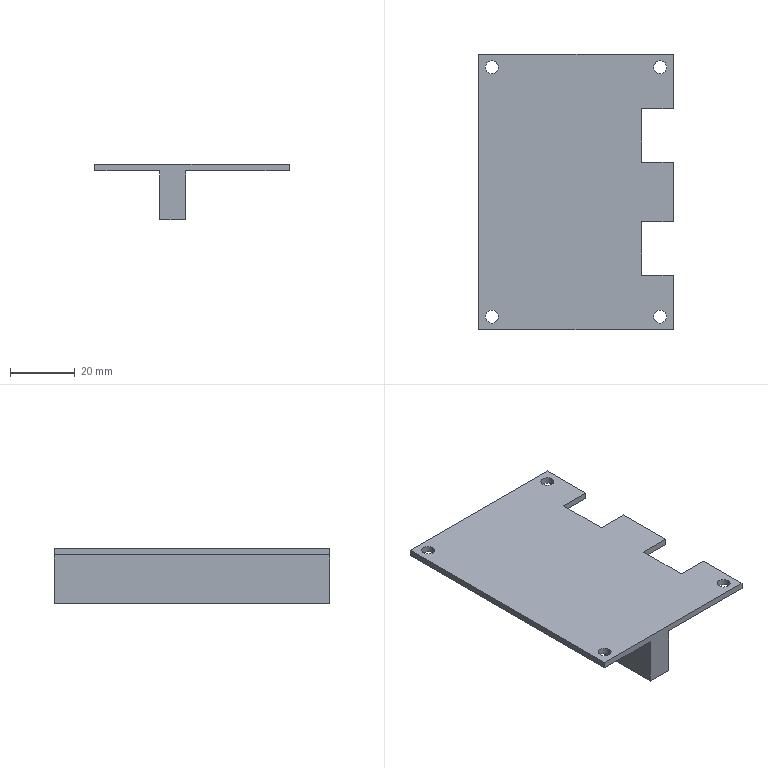Component | SolidWorks | WheelAssembly2-1_CoverPlate-1 | 1 solid | 26 faces | box 60 x 85 x 17 mm | volume 19659 mm3 | plane 18 | cylinder 8 | commonest cylinder face diameters 4 x8
STEP:
#1=CARTESIAN_POINT('',(-12.835,-1.516,-13.581));
#2=VERTEX_POINT('',#1);
#3=CARTESIAN_POINT('',(-12.677,-1.516,-13.581));
#4=VERTEX_POINT('',#3);
#5=CARTESIAN_POINT('',(-12.756,-1.516,-13.581));
#6=DIRECTION('',(0.,-0.,1.));
#7=DIRECTION('',(-1.,0.,0.));
#8=AXIS2_PLACEMENT_3D('',#5,#6,#7);
#9=CIRCLE('',#8,0.07874);
#10=EDGE_CURVE('',#2,#4,#9,.T.);
#11=ORIENTED_EDGE('',*,*,#10,.F.);
#12=CARTESIAN_POINT('',(-12.835,-1.516,-13.503));
#13=VERTEX_POINT('',#12);
#14=CARTESIAN_POINT('',(-12.835,-1.516,-13.581));
#15=DIRECTION('',(0.,-0.,1.));
#16=VECTOR('',#15,39.37);
#17=LINE('',#14,#16);
#18=EDGE_CURVE('',#2,#13,#17,.T.);
#19=ORIENTED_EDGE('',*,*,#18,.T.);
#20=CARTESIAN_POINT('',(-12.677,-1.516,-13.503));
#21=VERTEX_POINT('',#20);
#22=CARTESIAN_POINT('',(-12.756,-1.516,-13.503));
#23=DIRECTION('',(0.,-0.,1.));
#24=DIRECTION('',(-1.,0.,0.));
#25=AXIS2_PLACEMENT_3D('',#22,#23,#24);
#26=CIRCLE('',#25,0.07874);
#27=EDGE_CURVE('',#13,#21,#26,.T.);
#28=ORIENTED_EDGE('',*,*,#27,.T.);
#29=CARTESIAN_POINT('',(-12.677,-1.516,-13.581));
#30=DIRECTION('',(0.,-0.,1.));
#31=VECTOR('',#30,39.37);
#32=LINE('',#29,#31);
#33=EDGE_CURVE('',#4,#21,#32,.T.);
#34=ORIENTED_EDGE('',*,*,#33,.F.);
#35=EDGE_LOOP('',(#11,#19,#28,#34));
#36=FACE_OUTER_BOUND('',#35,.T.);
#37=CARTESIAN_POINT('',(-12.756,-1.516,-13.581));
#38=DIRECTION('',(0.,-0.,1.));
#39=DIRECTION('',(1.,0.,0.));
#40=AXIS2_PLACEMENT_3D('',#37,#38,#39);
#41=CYLINDRICAL_SURFACE('',#40,0.07874);
#42=ADVANCED_FACE('',(#36),#41,.F.);
#43=CARTESIAN_POINT('',(-12.835,1.516,-13.581));
#44=VERTEX_POINT('',#43);
#45=CARTESIAN_POINT('',(-12.677,1.516,-13.581));
#46=VERTEX_POINT('',#45);
#47=CARTESIAN_POINT('',(-12.756,1.516,-13.581));
#48=DIRECTION('',(0.,-0.,1.));
#49=DIRECTION('',(1.,0.,0.));
#50=AXIS2_PLACEMENT_3D('',#47,#48,#49);
#51=CIRCLE('',#50,0.07874);
#52=EDGE_CURVE('',#44,#46,#51,.T.);
#53=ORIENTED_EDGE('',*,*,#52,.F.);
#54=CARTESIAN_POINT('',(-12.835,1.516,-13.503));
#55=VERTEX_POINT('',#54);
#56=CARTESIAN_POINT('',(-12.835,1.516,-13.581));
#57=DIRECTION('',(0.,-0.,1.));
#58=VECTOR('',#57,39.37);
#59=LINE('',#56,#58);
#60=EDGE_CURVE('',#44,#55,#59,.T.);
#61=ORIENTED_EDGE('',*,*,#60,.T.);
#62=CARTESIAN_POINT('',(-12.677,1.516,-13.503));
#63=VERTEX_POINT('',#62);
#64=CARTESIAN_POINT('',(-12.756,1.516,-13.503));
#65=DIRECTION('',(0.,-0.,1.));
#66=DIRECTION('',(1.,0.,0.));
#67=AXIS2_PLACEMENT_3D('',#64,#65,#66);
#68=CIRCLE('',#67,0.07874);
#69=EDGE_CURVE('',#55,#63,#68,.T.);
#70=ORIENTED_EDGE('',*,*,#69,.T.);
#71=CARTESIAN_POINT('',(-12.677,1.516,-13.581));
#72=DIRECTION('',(0.,-0.,1.));
#73=VECTOR('',#72,39.37);
#74=LINE('',#71,#73);
#75=EDGE_CURVE('',#46,#63,#74,.T.);
#76=ORIENTED_EDGE('',*,*,#75,.F.);
#77=EDGE_LOOP('',(#53,#61,#70,#76));
#78=FACE_OUTER_BOUND('',#77,.T.);
#79=CARTESIAN_POINT('',(-12.756,1.516,-13.581));
#80=DIRECTION('',(0.,-0.,1.));
#81=DIRECTION('',(1.,0.,0.));
#82=AXIS2_PLACEMENT_3D('',#79,#80,#81);
#83=CYLINDRICAL_SURFACE('',#82,0.07874);
#84=ADVANCED_FACE('',(#78),#83,.F.);
#85=CARTESIAN_POINT('',(-14.882,1.516,-13.581));
#86=VERTEX_POINT('',#85);
#87=CARTESIAN_POINT('',(-14.724,1.516,-13.581));
#88=VERTEX_POINT('',#87);
#89=CARTESIAN_POINT('',(-14.803,1.516,-13.581));
#90=DIRECTION('',(0.,-0.,1.));
#91=DIRECTION('',(-1.,0.,0.));
#92=AXIS2_PLACEMENT_3D('',#89,#90,#91);
#93=CIRCLE('',#92,0.07874);
#94=EDGE_CURVE('',#86,#88,#93,.T.);
#95=ORIENTED_EDGE('',*,*,#94,.F.);
#96=CARTESIAN_POINT('',(-14.882,1.516,-13.503));
#97=VERTEX_POINT('',#96);
#98=CARTESIAN_POINT('',(-14.882,1.516,-13.581));
#99=DIRECTION('',(0.,-0.,1.));
#100=VECTOR('',#99,39.37);
#101=LINE('',#98,#100);
#102=EDGE_CURVE('',#86,#97,#101,.T.);
#103=ORIENTED_EDGE('',*,*,#102,.T.);
#104=CARTESIAN_POINT('',(-14.724,1.516,-13.503));
#105=VERTEX_POINT('',#104);
#106=CARTESIAN_POINT('',(-14.803,1.516,-13.503));
#107=DIRECTION('',(0.,-0.,1.));
#108=DIRECTION('',(-1.,0.,0.));
#109=AXIS2_PLACEMENT_3D('',#106,#107,#108);
#110=CIRCLE('',#109,0.07874);
#111=EDGE_CURVE('',#97,#105,#110,.T.);
#112=ORIENTED_EDGE('',*,*,#111,.T.);
#113=CARTESIAN_POINT('',(-14.724,1.516,-13.581));
#114=DIRECTION('',(0.,-0.,1.));
#115=VECTOR('',#114,39.37);
#116=LINE('',#113,#115);
#117=EDGE_CURVE('',#88,#105,#116,.T.);
#118=ORIENTED_EDGE('',*,*,#117,.F.);
#119=EDGE_LOOP('',(#95,#103,#112,#118));
#120=FACE_OUTER_BOUND('',#119,.T.);
#121=CARTESIAN_POINT('',(-14.803,1.516,-13.581));
#122=DIRECTION('',(0.,-0.,1.));
#123=DIRECTION('',(1.,0.,0.));
#124=AXIS2_PLACEMENT_3D('',#121,#122,#123);
#125=CYLINDRICAL_SURFACE('',#124,0.07874);
#126=ADVANCED_FACE('',(#120),#125,.F.);
#127=CARTESIAN_POINT('',(-14.882,-1.516,-13.581));
#128=VERTEX_POINT('',#127);
#129=CARTESIAN_POINT('',(-14.724,-1.516,-13.581));
#130=VERTEX_POINT('',#129);
#131=CARTESIAN_POINT('',(-14.803,-1.516,-13.581));
#132=DIRECTION('',(0.,-0.,1.));
#133=DIRECTION('',(1.,0.,0.));
#134=AXIS2_PLACEMENT_3D('',#131,#132,#133);
#135=CIRCLE('',#134,0.07874);
#136=EDGE_CURVE('',#128,#130,#135,.T.);
#137=ORIENTED_EDGE('',*,*,#136,.F.);
#138=CARTESIAN_POINT('',(-14.882,-1.516,-13.503));
#139=VERTEX_POINT('',#138);
#140=CARTESIAN_POINT('',(-14.882,-1.516,-13.581));
#141=DIRECTION('',(0.,-0.,1.));
#142=VECTOR('',#141,39.37);
#143=LINE('',#140,#142);
#144=EDGE_CURVE('',#128,#139,#143,.T.);
#145=ORIENTED_EDGE('',*,*,#144,.T.);
#146=CARTESIAN_POINT('',(-14.724,-1.516,-13.503));
#147=VERTEX_POINT('',#146);
#148=CARTESIAN_POINT('',(-14.803,-1.516,-13.503));
#149=DIRECTION('',(0.,-0.,1.));
#150=DIRECTION('',(1.,0.,0.));
#151=AXIS2_PLACEMENT_3D('',#148,#149,#150);
#152=CIRCLE('',#151,0.07874);
#153=EDGE_CURVE('',#139,#147,#152,.T.);
#154=ORIENTED_EDGE('',*,*,#153,.T.);
#155=CARTESIAN_POINT('',(-14.724,-1.516,-13.581));
#156=DIRECTION('',(0.,-0.,1.));
#157=VECTOR('',#156,39.37);
#158=LINE('',#155,#157);
#159=EDGE_CURVE('',#130,#147,#158,.T.);
#160=ORIENTED_EDGE('',*,*,#159,.F.);
#161=EDGE_LOOP('',(#137,#145,#154,#160));
#162=FACE_OUTER_BOUND('',#161,.T.);
#163=CARTESIAN_POINT('',(-14.803,-1.516,-13.581));
#164=DIRECTION('',(0.,-0.,1.));
#165=DIRECTION('',(1.,0.,0.));
#166=AXIS2_PLACEMENT_3D('',#163,#164,#165);
#167=CYLINDRICAL_SURFACE('',#166,0.07874);
#168=ADVANCED_FACE('',(#162),#167,.F.);
#169=CARTESIAN_POINT('',(-12.598,-0.3622,-13.581));
#170=VERTEX_POINT('',#169);
#171=CARTESIAN_POINT('',(-12.598,0.3622,-13.581));
#172=VERTEX_POINT('',#171);
#173=CARTESIAN_POINT('',(-12.598,-1.673,-13.581));
#174=DIRECTION('',(-0.,1.,0.));
#175=VECTOR('',#174,39.37);
#176=LINE('',#173,#175);
#177=EDGE_CURVE('',#170,#172,#176,.T.);
#178=ORIENTED_EDGE('',*,*,#177,.T.);
#179=CARTESIAN_POINT('',(-12.598,0.3622,-13.503));
#180=VERTEX_POINT('',#179);
#181=CARTESIAN_POINT('',(-12.598,0.3622,-13.503));
#182=DIRECTION('',(0.,-0.,1.));
#183=VECTOR('',#182,39.37);
#184=LINE('',#181,#183);
#185=EDGE_CURVE('',#172,#180,#184,.T.);
#186=ORIENTED_EDGE('',*,*,#185,.T.);
#187=CARTESIAN_POINT('',(-12.598,-0.3622,-13.503));
#188=VERTEX_POINT('',#187);
#189=CARTESIAN_POINT('',(-12.598,-1.673,-13.503));
#190=DIRECTION('',(-0.,1.,0.));
#191=VECTOR('',#190,39.37);
#192=LINE('',#189,#191);
#193=EDGE_CURVE('',#188,#180,#192,.T.);
#194=ORIENTED_EDGE('',*,*,#193,.F.);
#195=CARTESIAN_POINT('',(-12.598,-0.3622,-13.503));
#196=DIRECTION('',(-0.,0.,-1.));
#197=VECTOR('',#196,39.37);
#198=LINE('',#195,#197);
#199=EDGE_CURVE('',#188,#170,#198,.T.);
#200=ORIENTED_EDGE('',*,*,#199,.T.);
#201=EDGE_LOOP('',(#178,#186,#194,#200));
#202=FACE_OUTER_BOUND('',#201,.T.);
#203=CARTESIAN_POINT('',(-12.598,-1.673,-13.503));
#204=DIRECTION('',(-1.,-0.,0.));
#205=DIRECTION('',(0.,-1.,-0.));
#206=AXIS2_PLACEMENT_3D('',#203,#204,#205);
#207=PLANE('',#206);
#208=ADVANCED_FACE('',(#202),#207,.F.);
#209=CARTESIAN_POINT('',(-12.598,-1.673,-13.581));
#210=VERTEX_POINT('',#209);
#211=CARTESIAN_POINT('',(-12.598,-1.012,-13.581));
#212=VERTEX_POINT('',#211);
#213=CARTESIAN_POINT('',(-12.598,-1.673,-13.581));
#214=DIRECTION('',(-0.,1.,0.));
#215=VECTOR('',#214,39.37);
#216=LINE('',#213,#215);
#217=EDGE_CURVE('',#210,#212,#216,.T.);
#218=ORIENTED_EDGE('',*,*,#217,.T.);
#219=CARTESIAN_POINT('',(-12.598,-1.012,-13.503));
#220=VERTEX_POINT('',#219);
#221=CARTESIAN_POINT('',(-12.598,-1.012,-13.503));
#222=DIRECTION('',(0.,-0.,1.));
#223=VECTOR('',#222,39.37);
#224=LINE('',#221,#223);
#225=EDGE_CURVE('',#212,#220,#224,.T.);
#226=ORIENTED_EDGE('',*,*,#225,.T.);
#227=CARTESIAN_POINT('',(-12.598,-1.673,-13.503));
#228=VERTEX_POINT('',#227);
#229=CARTESIAN_POINT('',(-12.598,-1.673,-13.503));
#230=DIRECTION('',(-0.,1.,0.));
#231=VECTOR('',#230,39.37);
#232=LINE('',#229,#231);
#233=EDGE_CURVE('',#228,#220,#232,.T.);
#234=ORIENTED_EDGE('',*,*,#233,.F.);
#235=CARTESIAN_POINT('',(-12.598,-1.673,-13.503));
#236=DIRECTION('',(-0.,0.,-1.));
#237=VECTOR('',#236,39.37);
#238=LINE('',#235,#237);
#239=EDGE_CURVE('',#228,#210,#238,.T.);
#240=ORIENTED_EDGE('',*,*,#239,.T.);
#241=EDGE_LOOP('',(#218,#226,#234,#240));
#242=FACE_OUTER_BOUND('',#241,.T.);
#243=CARTESIAN_POINT('',(-12.598,-1.673,-13.503));
#244=DIRECTION('',(-1.,-0.,0.));
#245=DIRECTION('',(0.,-1.,-0.));
#246=AXIS2_PLACEMENT_3D('',#243,#244,#245);
#247=PLANE('',#246);
#248=ADVANCED_FACE('',(#242),#247,.F.);
#249=CARTESIAN_POINT('',(-14.803,-1.516,-13.581));
#250=DIRECTION('',(0.,-0.,1.));
#251=DIRECTION('',(1.,0.,0.));
#252=AXIS2_PLACEMENT_3D('',#249,#250,#251);
#253=CIRCLE('',#252,0.07874);
#254=EDGE_CURVE('',#130,#128,#253,.T.);
#255=ORIENTED_EDGE('',*,*,#254,.T.);
#256=ORIENTED_EDGE('',*,*,#136,.T.);
#257=EDGE_LOOP('',(#255,#256));
#258=FACE_BOUND('',#257,.T.);
#259=CARTESIAN_POINT('',(-14.803,1.516,-13.581));
#260=DIRECTION('',(0.,-0.,1.));
#261=DIRECTION('',(-1.,0.,0.));
#262=AXIS2_PLACEMENT_3D('',#259,#260,#261);
#263=CIRCLE('',#262,0.07874);
#264=EDGE_CURVE('',#88,#86,#263,.T.);
#265=ORIENTED_EDGE('',*,*,#264,.T.);
#266=ORIENTED_EDGE('',*,*,#94,.T.);
#267=EDGE_LOOP('',(#265,#266));
#268=FACE_BOUND('',#267,.T.);
#269=CARTESIAN_POINT('',(-14.173,1.673,-13.581));
#270=VERTEX_POINT('',#269);
#271=CARTESIAN_POINT('',(-14.961,1.673,-13.581));
#272=VERTEX_POINT('',#271);
#273=CARTESIAN_POINT('',(-14.961,1.673,-13.581));
#274=DIRECTION('',(-1.,-0.,0.));
#275=VECTOR('',#274,39.37);
#276=LINE('',#273,#275);
#277=EDGE_CURVE('',#270,#272,#276,.T.);
#278=ORIENTED_EDGE('',*,*,#277,.F.);
#279=CARTESIAN_POINT('',(-14.173,-1.673,-13.581));
#280=VERTEX_POINT('',#279);
#281=CARTESIAN_POINT('',(-14.173,0.,-13.581));
#282=DIRECTION('',(0.,-1.,-0.));
#283=VECTOR('',#282,39.37);
#284=LINE('',#281,#283);
#285=EDGE_CURVE('',#270,#280,#284,.T.);
#286=ORIENTED_EDGE('',*,*,#285,.T.);
#287=CARTESIAN_POINT('',(-14.961,-1.673,-13.581));
#288=VERTEX_POINT('',#287);
#289=CARTESIAN_POINT('',(-14.961,-1.673,-13.581));
#290=DIRECTION('',(1.,0.,-0.));
#291=VECTOR('',#290,39.37);
#292=LINE('',#289,#291);
#293=EDGE_CURVE('',#288,#280,#292,.T.);
#294=ORIENTED_EDGE('',*,*,#293,.F.);
#295=CARTESIAN_POINT('',(-14.961,-1.673,-13.581));
#296=DIRECTION('',(0.,-1.,-0.));
#297=VECTOR('',#296,39.37);
#298=LINE('',#295,#297);
#299=EDGE_CURVE('',#272,#288,#298,.T.);
#300=ORIENTED_EDGE('',*,*,#299,.F.);
#301=EDGE_LOOP('',(#278,#286,#294,#300));
#302=FACE_OUTER_BOUND('',#301,.T.);
#303=CARTESIAN_POINT('',(-13.78,0.,-13.581));
#304=DIRECTION('',(0.,-0.,1.));
#305=DIRECTION('',(1.,0.,-0.));
#306=AXIS2_PLACEMENT_3D('',#303,#304,#305);
#307=PLANE('',#306);
#308=ADVANCED_FACE('',(#258,#268,#302),#307,.F.);
#309=CARTESIAN_POINT('',(-14.173,1.673,-14.172));
#310=VERTEX_POINT('',#309);
#311=CARTESIAN_POINT('',(-14.173,1.673,-14.172));
#312=DIRECTION('',(0.,-0.,1.));
#313=VECTOR('',#312,39.37);
#314=LINE('',#311,#313);
#315=EDGE_CURVE('',#310,#270,#314,.T.);
#316=ORIENTED_EDGE('',*,*,#315,.T.);
#317=ORIENTED_EDGE('',*,*,#277,.T.);
#318=CARTESIAN_POINT('',(-14.961,1.673,-13.503));
#319=VERTEX_POINT('',#318);
#320=CARTESIAN_POINT('',(-14.961,1.673,-13.503));
#321=DIRECTION('',(-0.,0.,-1.));
#322=VECTOR('',#321,39.37);
#323=LINE('',#320,#322);
#324=EDGE_CURVE('',#319,#272,#323,.T.);
#325=ORIENTED_EDGE('',*,*,#324,.F.);
#326=CARTESIAN_POINT('',(-12.598,1.673,-13.503));
#327=VERTEX_POINT('',#326);
#328=CARTESIAN_POINT('',(-14.961,1.673,-13.503));
#329=DIRECTION('',(-1.,-0.,0.));
#330=VECTOR('',#329,39.37);
#331=LINE('',#328,#330);
#332=EDGE_CURVE('',#327,#319,#331,.T.);
#333=ORIENTED_EDGE('',*,*,#332,.F.);
#334=CARTESIAN_POINT('',(-12.598,1.673,-13.581));
#335=VERTEX_POINT('',#334);
#336=CARTESIAN_POINT('',(-12.598,1.673,-13.503));
#337=DIRECTION('',(-0.,0.,-1.));
#338=VECTOR('',#337,39.37);
#339=LINE('',#336,#338);
#340=EDGE_CURVE('',#327,#335,#339,.T.);
#341=ORIENTED_EDGE('',*,*,#340,.T.);
#342=CARTESIAN_POINT('',(-13.858,1.673,-13.581));
#343=VERTEX_POINT('',#342);
#344=CARTESIAN_POINT('',(-14.961,1.673,-13.581));
#345=DIRECTION('',(-1.,-0.,0.));
#346=VECTOR('',#345,39.37);
#347=LINE('',#344,#346);
#348=EDGE_CURVE('',#335,#343,#347,.T.);
#349=ORIENTED_EDGE('',*,*,#348,.T.);
#350=CARTESIAN_POINT('',(-13.858,1.673,-14.172));
#351=VERTEX_POINT('',#350);
#352=CARTESIAN_POINT('',(-13.858,1.673,-14.172));
#353=DIRECTION('',(-0.,0.,-1.));
#354=VECTOR('',#353,39.37);
#355=LINE('',#352,#354);
#356=EDGE_CURVE('',#343,#351,#355,.T.);
#357=ORIENTED_EDGE('',*,*,#356,.T.);
#358=CARTESIAN_POINT('',(-14.173,1.673,-14.172));
#359=DIRECTION('',(-1.,-0.,0.));
#360=VECTOR('',#359,39.37);
#361=LINE('',#358,#360);
#362=EDGE_CURVE('',#351,#310,#361,.T.);
#363=ORIENTED_EDGE('',*,*,#362,.T.);
#364=EDGE_LOOP('',(#316,#317,#325,#333,#341,#349,#357,#363));
#365=FACE_OUTER_BOUND('',#364,.T.);
#366=CARTESIAN_POINT('',(-14.961,1.673,-13.503));
#367=DIRECTION('',(0.,-1.,-0.));
#368=DIRECTION('',(1.,0.,-0.));
#369=AXIS2_PLACEMENT_3D('',#366,#367,#368);
#370=PLANE('',#369);
#371=ADVANCED_FACE('',(#365),#370,.F.);
#372=ORIENTED_EDGE('',*,*,#299,.T.);
#373=CARTESIAN_POINT('',(-14.961,-1.673,-13.503));
#374=VERTEX_POINT('',#373);
#375=CARTESIAN_POINT('',(-14.961,-1.673,-13.503));
#376=DIRECTION('',(-0.,0.,-1.));
#377=VECTOR('',#376,39.37);
#378=LINE('',#375,#377);
#379=EDGE_CURVE('',#374,#288,#378,.T.);
#380=ORIENTED_EDGE('',*,*,#379,.F.);
#381=CARTESIAN_POINT('',(-14.961,-1.673,-13.503));
#382=DIRECTION('',(0.,-1.,-0.));
#383=VECTOR('',#382,39.37);
#384=LINE('',#381,#383);
#385=EDGE_CURVE('',#319,#374,#384,.T.);
#386=ORIENTED_EDGE('',*,*,#385,.F.);
#387=ORIENTED_EDGE('',*,*,#324,.T.);
#388=EDGE_LOOP('',(#372,#380,#386,#387));
#389=FACE_OUTER_BOUND('',#388,.T.);
#390=CARTESIAN_POINT('',(-14.961,-1.673,-13.503));
#391=DIRECTION('',(1.,0.,-0.));
#392=DIRECTION('',(-0.,1.,0.));
#393=AXIS2_PLACEMENT_3D('',#390,#391,#392);
#394=PLANE('',#393);
#395=ADVANCED_FACE('',(#389),#394,.F.);
#396=ORIENTED_EDGE('',*,*,#293,.T.);
#397=CARTESIAN_POINT('',(-14.173,-1.673,-14.172));
#398=VERTEX_POINT('',#397);
#399=CARTESIAN_POINT('',(-14.173,-1.673,-14.172));
#400=DIRECTION('',(-0.,0.,-1.));
#401=VECTOR('',#400,39.37);
#402=LINE('',#399,#401);
#403=EDGE_CURVE('',#280,#398,#402,.T.);
#404=ORIENTED_EDGE('',*,*,#403,.T.);
#405=CARTESIAN_POINT('',(-13.858,-1.673,-14.172));
#406=VERTEX_POINT('',#405);
#407=CARTESIAN_POINT('',(-14.173,-1.673,-14.172));
#408=DIRECTION('',(1.,0.,-0.));
#409=VECTOR('',#408,39.37);
#410=LINE('',#407,#409);
#411=EDGE_CURVE('',#398,#406,#410,.T.);
#412=ORIENTED_EDGE('',*,*,#411,.T.);
#413=CARTESIAN_POINT('',(-13.858,-1.673,-13.581));
#414=VERTEX_POINT('',#413);
#415=CARTESIAN_POINT('',(-13.858,-1.673,-14.172));
#416=DIRECTION('',(0.,-0.,1.));
#417=VECTOR('',#416,39.37);
#418=LINE('',#415,#417);
#419=EDGE_CURVE('',#406,#414,#418,.T.);
#420=ORIENTED_EDGE('',*,*,#419,.T.);
#421=CARTESIAN_POINT('',(-14.961,-1.673,-13.581));
#422=DIRECTION('',(1.,0.,-0.));
#423=VECTOR('',#422,39.37);
#424=LINE('',#421,#423);
#425=EDGE_CURVE('',#414,#210,#424,.T.);
#426=ORIENTED_EDGE('',*,*,#425,.T.);
#427=ORIENTED_EDGE('',*,*,#239,.F.);
#428=CARTESIAN_POINT('',(-14.961,-1.673,-13.503));
#429=DIRECTION('',(1.,0.,-0.));
#430=VECTOR('',#429,39.37);
#431=LINE('',#428,#430);
#432=EDGE_CURVE('',#374,#228,#431,.T.);
#433=ORIENTED_EDGE('',*,*,#432,.F.);
#434=ORIENTED_EDGE('',*,*,#379,.T.);
#435=EDGE_LOOP('',(#396,#404,#412,#420,#426,#427,#433,#434));
#436=FACE_OUTER_BOUND('',#435,.T.);
#437=CARTESIAN_POINT('',(-14.961,-1.673,-13.503));
#438=DIRECTION('',(-0.,1.,0.));
#439=DIRECTION('',(-1.,-0.,0.));
#440=AXIS2_PLACEMENT_3D('',#437,#438,#439);
#441=PLANE('',#440);
#442=ADVANCED_FACE('',(#436),#441,.F.);
#443=CARTESIAN_POINT('',(-12.598,1.012,-13.503));
#444=VERTEX_POINT('',#443);
#445=CARTESIAN_POINT('',(-12.598,-1.673,-13.503));
#446=DIRECTION('',(-0.,1.,0.));
#447=VECTOR('',#446,39.37);
#448=LINE('',#445,#447);
#449=EDGE_CURVE('',#444,#327,#448,.T.);
#450=ORIENTED_EDGE('',*,*,#449,.F.);
#451=CARTESIAN_POINT('',(-12.598,1.012,-13.581));
#452=VERTEX_POINT('',#451);
#453=CARTESIAN_POINT('',(-12.598,1.012,-13.503));
#454=DIRECTION('',(-0.,0.,-1.));
#455=VECTOR('',#454,39.37);
#456=LINE('',#453,#455);
#457=EDGE_CURVE('',#444,#452,#456,.T.);
#458=ORIENTED_EDGE('',*,*,#457,.T.);
#459=CARTESIAN_POINT('',(-12.598,-1.673,-13.581));
#460=DIRECTION('',(-0.,1.,0.));
#461=VECTOR('',#460,39.37);
#462=LINE('',#459,#461);
#463=EDGE_CURVE('',#452,#335,#462,.T.);
#464=ORIENTED_EDGE('',*,*,#463,.T.);
#465=ORIENTED_EDGE('',*,*,#340,.F.);
#466=EDGE_LOOP('',(#450,#458,#464,#465));
#467=FACE_OUTER_BOUND('',#466,.T.);
#468=CARTESIAN_POINT('',(-12.598,-1.673,-13.503));
#469=DIRECTION('',(-1.,-0.,0.));
#470=DIRECTION('',(0.,-1.,-0.));
#471=AXIS2_PLACEMENT_3D('',#468,#469,#470);
#472=PLANE('',#471);
#473=ADVANCED_FACE('',(#467),#472,.F.);
#474=CARTESIAN_POINT('',(-12.98,0.3622,-13.503));
#475=VERTEX_POINT('',#474);
#476=CARTESIAN_POINT('',(-12.98,0.3622,-13.503));
#477=DIRECTION('',(1.,0.,-0.));
#478=VECTOR('',#477,39.37);
#479=LINE('',#476,#478);
#480=EDGE_CURVE('',#475,#180,#479,.T.);
#481=ORIENTED_EDGE('',*,*,#480,.F.);
#482=CARTESIAN_POINT('',(-12.98,1.012,-13.503));
#483=VERTEX_POINT('',#482);
#484=CARTESIAN_POINT('',(-12.98,0.3622,-13.503));
#485=DIRECTION('',(0.,-1.,-0.));
#486=VECTOR('',#485,39.37);
#487=LINE('',#484,#486);
#488=EDGE_CURVE('',#483,#475,#487,.T.);
#489=ORIENTED_EDGE('',*,*,#488,.F.);
#490=CARTESIAN_POINT('',(-12.98,1.012,-13.503));
#491=DIRECTION('',(-1.,-0.,0.));
#492=VECTOR('',#491,39.37);
#493=LINE('',#490,#492);
#494=EDGE_CURVE('',#444,#483,#493,.T.);
#495=ORIENTED_EDGE('',*,*,#494,.F.);
#496=ORIENTED_EDGE('',*,*,#449,.T.);
#497=ORIENTED_EDGE('',*,*,#332,.T.);
#498=ORIENTED_EDGE('',*,*,#385,.T.);
#499=ORIENTED_EDGE('',*,*,#432,.T.);
#500=ORIENTED_EDGE('',*,*,#233,.T.);
#501=CARTESIAN_POINT('',(-12.98,-1.012,-13.503));
#502=VERTEX_POINT('',#501);
#503=CARTESIAN_POINT('',(-12.98,-1.012,-13.503));
#504=DIRECTION('',(1.,0.,-0.));
#505=VECTOR('',#504,39.37);
#506=LINE('',#503,#505);
#507=EDGE_CURVE('',#502,#220,#506,.T.);
#508=ORIENTED_EDGE('',*,*,#507,.F.);
#509=CARTESIAN_POINT('',(-12.98,-0.3622,-13.503));
#510=VERTEX_POINT('',#509);
#511=CARTESIAN_POINT('',(-12.98,-1.012,-13.503));
#512=DIRECTION('',(0.,-1.,-0.));
#513=VECTOR('',#512,39.37);
#514=LINE('',#511,#513);
#515=EDGE_CURVE('',#510,#502,#514,.T.);
#516=ORIENTED_EDGE('',*,*,#515,.F.);
#517=CARTESIAN_POINT('',(-12.98,-0.3622,-13.503));
#518=DIRECTION('',(-1.,-0.,0.));
#519=VECTOR('',#518,39.37);
#520=LINE('',#517,#519);
#521=EDGE_CURVE('',#188,#510,#520,.T.);
#522=ORIENTED_EDGE('',*,*,#521,.F.);
#523=ORIENTED_EDGE('',*,*,#193,.T.);
#524=EDGE_LOOP('',(#481,#489,#495,#496,#497,#498,#499,#500,#508,#516,#522,#523));
#525=FACE_OUTER_BOUND('',#524,.T.);
#526=CARTESIAN_POINT('',(-12.756,-1.516,-13.503));
#527=DIRECTION('',(0.,-0.,1.));
#528=DIRECTION('',(-1.,0.,0.));
#529=AXIS2_PLACEMENT_3D('',#526,#527,#528);
#530=CIRCLE('',#529,0.07874);
#531=EDGE_CURVE('',#21,#13,#530,.T.);
#532=ORIENTED_EDGE('',*,*,#531,.F.);
#533=ORIENTED_EDGE('',*,*,#27,.F.);
#534=EDGE_LOOP('',(#532,#533));
#535=FACE_BOUND('',#534,.T.);
#536=CARTESIAN_POINT('',(-12.756,1.516,-13.503));
#537=DIRECTION('',(0.,-0.,1.));
#538=DIRECTION('',(1.,0.,0.));
#539=AXIS2_PLACEMENT_3D('',#536,#537,#538);
#540=CIRCLE('',#539,0.07874);
#541=EDGE_CURVE('',#63,#55,#540,.T.);
#542=ORIENTED_EDGE('',*,*,#541,.F.);
#543=ORIENTED_EDGE('',*,*,#69,.F.);
#544=EDGE_LOOP('',(#542,#543));
#545=FACE_BOUND('',#544,.T.);
#546=CARTESIAN_POINT('',(-14.803,1.516,-13.503));
#547=DIRECTION('',(0.,-0.,1.));
#548=DIRECTION('',(-1.,0.,0.));
#549=AXIS2_PLACEMENT_3D('',#546,#547,#548);
#550=CIRCLE('',#549,0.07874);
#551=EDGE_CURVE('',#105,#97,#550,.T.);
#552=ORIENTED_EDGE('',*,*,#551,.F.);
#553=ORIENTED_EDGE('',*,*,#111,.F.);
#554=EDGE_LOOP('',(#552,#553));
#555=FACE_BOUND('',#554,.T.);
#556=CARTESIAN_POINT('',(-14.803,-1.516,-13.503));
#557=DIRECTION('',(0.,-0.,1.));
#558=DIRECTION('',(1.,0.,0.));
#559=AXIS2_PLACEMENT_3D('',#556,#557,#558);
#560=CIRCLE('',#559,0.07874);
#561=EDGE_CURVE('',#147,#139,#560,.T.);
#562=ORIENTED_EDGE('',*,*,#561,.F.);
#563=ORIENTED_EDGE('',*,*,#153,.F.);
#564=EDGE_LOOP('',(#562,#563));
#565=FACE_BOUND('',#564,.T.);
#566=CARTESIAN_POINT('',(-13.78,0.,-13.503));
#567=DIRECTION('',(0.,-0.,1.));
#568=DIRECTION('',(1.,0.,-0.));
#569=AXIS2_PLACEMENT_3D('',#566,#567,#568);
#570=PLANE('',#569);
#571=ADVANCED_FACE('',(#525,#535,#545,#555,#565),#570,.T.);
#572=CARTESIAN_POINT('',(-12.756,-1.516,-13.581));
#573=DIRECTION('',(0.,-0.,1.));
#574=DIRECTION('',(-1.,0.,0.));
#575=AXIS2_PLACEMENT_3D('',#572,#573,#574);
#576=CIRCLE('',#575,0.07874);
#577=EDGE_CURVE('',#4,#2,#576,.T.);
#578=ORIENTED_EDGE('',*,*,#577,.T.);
#579=ORIENTED_EDGE('',*,*,#10,.T.);
#580=EDGE_LOOP('',(#578,#579));
#581=FACE_BOUND('',#580,.T.);
#582=CARTESIAN_POINT('',(-12.756,1.516,-13.581));
#583=DIRECTION('',(0.,-0.,1.));
#584=DIRECTION('',(1.,0.,0.));
#585=AXIS2_PLACEMENT_3D('',#582,#583,#584);
#586=CIRCLE('',#585,0.07874);
#587=EDGE_CURVE('',#46,#44,#586,.T.);
#588=ORIENTED_EDGE('',*,*,#587,.T.);
#589=ORIENTED_EDGE('',*,*,#52,.T.);
#590=EDGE_LOOP('',(#588,#589));
#591=FACE_BOUND('',#590,.T.);
#592=CARTESIAN_POINT('',(-12.98,1.012,-13.581));
#593=VERTEX_POINT('',#592);
#594=CARTESIAN_POINT('',(-12.98,0.3622,-13.581));
#595=VERTEX_POINT('',#594);
#596=CARTESIAN_POINT('',(-12.98,0.,-13.581));
#597=DIRECTION('',(0.,-1.,-0.));
#598=VECTOR('',#597,39.37);
#599=LINE('',#596,#598);
#600=EDGE_CURVE('',#593,#595,#599,.T.);
#601=ORIENTED_EDGE('',*,*,#600,.T.);
#602=CARTESIAN_POINT('',(-13.78,0.3622,-13.581));
#603=DIRECTION('',(1.,0.,-0.));
#604=VECTOR('',#603,39.37);
#605=LINE('',#602,#604);
#606=EDGE_CURVE('',#595,#172,#605,.T.);
#607=ORIENTED_EDGE('',*,*,#606,.T.);
#608=ORIENTED_EDGE('',*,*,#177,.F.);
#609=CARTESIAN_POINT('',(-12.98,-0.3622,-13.581));
#610=VERTEX_POINT('',#609);
#611=CARTESIAN_POINT('',(-13.78,-0.3622,-13.581));
#612=DIRECTION('',(-1.,-0.,0.));
#613=VECTOR('',#612,39.37);
#614=LINE('',#611,#613);
#615=EDGE_CURVE('',#170,#610,#614,.T.);
#616=ORIENTED_EDGE('',*,*,#615,.T.);
#617=CARTESIAN_POINT('',(-12.98,-1.012,-13.581));
#618=VERTEX_POINT('',#617);
#619=CARTESIAN_POINT('',(-12.98,0.,-13.581));
#620=DIRECTION('',(0.,-1.,-0.));
#621=VECTOR('',#620,39.37);
#622=LINE('',#619,#621);
#623=EDGE_CURVE('',#610,#618,#622,.T.);
#624=ORIENTED_EDGE('',*,*,#623,.T.);
#625=CARTESIAN_POINT('',(-13.78,-1.012,-13.581));
#626=DIRECTION('',(1.,0.,-0.));
#627=VECTOR('',#626,39.37);
#628=LINE('',#625,#627);
#629=EDGE_CURVE('',#618,#212,#628,.T.);
#630=ORIENTED_EDGE('',*,*,#629,.T.);
#631=ORIENTED_EDGE('',*,*,#217,.F.);
#632=ORIENTED_EDGE('',*,*,#425,.F.);
#633=CARTESIAN_POINT('',(-13.858,0.,-13.581));
#634=DIRECTION('',(-0.,1.,0.));
#635=VECTOR('',#634,39.37);
#636=LINE('',#633,#635);
#637=EDGE_CURVE('',#414,#343,#636,.T.);
#638=ORIENTED_EDGE('',*,*,#637,.T.);
#639=ORIENTED_EDGE('',*,*,#348,.F.);
#640=ORIENTED_EDGE('',*,*,#463,.F.);
#641=CARTESIAN_POINT('',(-13.78,1.012,-13.581));
#642=DIRECTION('',(-1.,-0.,0.));
#643=VECTOR('',#642,39.37);
#644=LINE('',#641,#643);
#645=EDGE_CURVE('',#452,#593,#644,.T.);
#646=ORIENTED_EDGE('',*,*,#645,.T.);
#647=EDGE_LOOP('',(#601,#607,#608,#616,#624,#630,#631,#632,#638,#639,#640,#646));
#648=FACE_OUTER_BOUND('',#647,.T.);
#649=CARTESIAN_POINT('',(-13.78,0.,-13.581));
#650=DIRECTION('',(0.,-0.,1.));
#651=DIRECTION('',(1.,0.,-0.));
#652=AXIS2_PLACEMENT_3D('',#649,#650,#651);
#653=PLANE('',#652);
#654=ADVANCED_FACE('',(#581,#591,#648),#653,.F.);
#655=ORIENTED_EDGE('',*,*,#144,.F.);
#656=ORIENTED_EDGE('',*,*,#254,.F.);
#657=ORIENTED_EDGE('',*,*,#159,.T.);
#658=ORIENTED_EDGE('',*,*,#561,.T.);
#659=EDGE_LOOP('',(#655,#656,#657,#658));
#660=FACE_OUTER_BOUND('',#659,.T.);
#661=CARTESIAN_POINT('',(-14.803,-1.516,-13.581));
#662=DIRECTION('',(0.,-0.,1.));
#663=DIRECTION('',(1.,0.,0.));
#664=AXIS2_PLACEMENT_3D('',#661,#662,#663);
#665=CYLINDRICAL_SURFACE('',#664,0.07874);
#666=ADVANCED_FACE('',(#660),#665,.F.);
#667=ORIENTED_EDGE('',*,*,#102,.F.);
#668=ORIENTED_EDGE('',*,*,#264,.F.);
#669=ORIENTED_EDGE('',*,*,#117,.T.);
#670=ORIENTED_EDGE('',*,*,#551,.T.);
#671=EDGE_LOOP('',(#667,#668,#669,#670));
#672=FACE_OUTER_BOUND('',#671,.T.);
#673=CARTESIAN_POINT('',(-14.803,1.516,-13.581));
#674=DIRECTION('',(0.,-0.,1.));
#675=DIRECTION('',(1.,0.,0.));
#676=AXIS2_PLACEMENT_3D('',#673,#674,#675);
#677=CYLINDRICAL_SURFACE('',#676,0.07874);
#678=ADVANCED_FACE('',(#672),#677,.F.);
#679=ORIENTED_EDGE('',*,*,#60,.F.);
#680=ORIENTED_EDGE('',*,*,#587,.F.);
#681=ORIENTED_EDGE('',*,*,#75,.T.);
#682=ORIENTED_EDGE('',*,*,#541,.T.);
#683=EDGE_LOOP('',(#679,#680,#681,#682));
#684=FACE_OUTER_BOUND('',#683,.T.);
#685=CARTESIAN_POINT('',(-12.756,1.516,-13.581));
#686=DIRECTION('',(0.,-0.,1.));
#687=DIRECTION('',(1.,0.,0.));
#688=AXIS2_PLACEMENT_3D('',#685,#686,#687);
#689=CYLINDRICAL_SURFACE('',#688,0.07874);
#690=ADVANCED_FACE('',(#684),#689,.F.);
#691=ORIENTED_EDGE('',*,*,#18,.F.);
#692=ORIENTED_EDGE('',*,*,#577,.F.);
#693=ORIENTED_EDGE('',*,*,#33,.T.);
#694=ORIENTED_EDGE('',*,*,#531,.T.);
#695=EDGE_LOOP('',(#691,#692,#693,#694));
#696=FACE_OUTER_BOUND('',#695,.T.);
#697=CARTESIAN_POINT('',(-12.756,-1.516,-13.581));
#698=DIRECTION('',(0.,-0.,1.));
#699=DIRECTION('',(1.,0.,0.));
#700=AXIS2_PLACEMENT_3D('',#697,#698,#699);
#701=CYLINDRICAL_SURFACE('',#700,0.07874);
#702=ADVANCED_FACE('',(#696),#701,.F.);
#703=ORIENTED_EDGE('',*,*,#285,.F.);
#704=ORIENTED_EDGE('',*,*,#315,.F.);
#705=CARTESIAN_POINT('',(-14.173,2.343,-14.172));
#706=DIRECTION('',(0.,-1.,-0.));
#707=VECTOR('',#706,39.37);
#708=LINE('',#705,#707);
#709=EDGE_CURVE('',#310,#398,#708,.T.);
#710=ORIENTED_EDGE('',*,*,#709,.T.);
#711=ORIENTED_EDGE('',*,*,#403,.F.);
#712=EDGE_LOOP('',(#703,#704,#710,#711));
#713=FACE_OUTER_BOUND('',#712,.T.);
#714=CARTESIAN_POINT('',(-14.173,2.343,-14.172));
#715=DIRECTION('',(-1.,-0.,0.));
#716=DIRECTION('',(0.,-1.,-0.));
#717=AXIS2_PLACEMENT_3D('',#714,#715,#716);
#718=PLANE('',#717);
#719=ADVANCED_FACE('',(#713),#718,.T.);
#720=ORIENTED_EDGE('',*,*,#637,.F.);
#721=ORIENTED_EDGE('',*,*,#419,.F.);
#722=CARTESIAN_POINT('',(-13.858,2.343,-14.172));
#723=DIRECTION('',(0.,-1.,-0.));
#724=VECTOR('',#723,39.37);
#725=LINE('',#722,#724);
#726=EDGE_CURVE('',#351,#406,#725,.T.);
#727=ORIENTED_EDGE('',*,*,#726,.F.);
#728=ORIENTED_EDGE('',*,*,#356,.F.);
#729=EDGE_LOOP('',(#720,#721,#727,#728));
#730=FACE_OUTER_BOUND('',#729,.T.);
#731=CARTESIAN_POINT('',(-13.858,2.343,-14.172));
#732=DIRECTION('',(1.,0.,-0.));
#733=DIRECTION('',(-0.,0.,-1.));
#734=AXIS2_PLACEMENT_3D('',#731,#732,#733);
#735=PLANE('',#734);
#736=ADVANCED_FACE('',(#730),#735,.T.);
#737=ORIENTED_EDGE('',*,*,#362,.F.);
#738=ORIENTED_EDGE('',*,*,#726,.T.);
#739=ORIENTED_EDGE('',*,*,#411,.F.);
#740=ORIENTED_EDGE('',*,*,#709,.F.);
#741=EDGE_LOOP('',(#737,#738,#739,#740));
#742=FACE_OUTER_BOUND('',#741,.T.);
#743=CARTESIAN_POINT('',(-14.173,2.343,-14.172));
#744=DIRECTION('',(-0.,0.,-1.));
#745=DIRECTION('',(-1.,-0.,0.));
#746=AXIS2_PLACEMENT_3D('',#743,#744,#745);
#747=PLANE('',#746);
#748=ADVANCED_FACE('',(#742),#747,.T.);
#749=ORIENTED_EDGE('',*,*,#629,.F.);
#750=CARTESIAN_POINT('',(-12.98,-1.012,-14.172));
#751=DIRECTION('',(0.,-0.,1.));
#752=VECTOR('',#751,39.37);
#753=LINE('',#750,#752);
#754=EDGE_CURVE('',#618,#502,#753,.T.);
#755=ORIENTED_EDGE('',*,*,#754,.T.);
#756=ORIENTED_EDGE('',*,*,#507,.T.);
#757=ORIENTED_EDGE('',*,*,#225,.F.);
#758=EDGE_LOOP('',(#749,#755,#756,#757));
#759=FACE_OUTER_BOUND('',#758,.T.);
#760=CARTESIAN_POINT('',(-12.98,-1.012,-14.172));
#761=DIRECTION('',(0.,-1.,-0.));
#762=DIRECTION('',(1.,0.,-0.));
#763=AXIS2_PLACEMENT_3D('',#760,#761,#762);
#764=PLANE('',#763);
#765=ADVANCED_FACE('',(#759),#764,.F.);
#766=CARTESIAN_POINT('',(-12.98,-0.3622,-14.172));
#767=DIRECTION('',(0.,-0.,1.));
#768=VECTOR('',#767,39.37);
#769=LINE('',#766,#768);
#770=EDGE_CURVE('',#610,#510,#769,.T.);
#771=ORIENTED_EDGE('',*,*,#770,.T.);
#772=ORIENTED_EDGE('',*,*,#515,.T.);
#773=ORIENTED_EDGE('',*,*,#754,.F.);
#774=ORIENTED_EDGE('',*,*,#623,.F.);
#775=EDGE_LOOP('',(#771,#772,#773,#774));
#776=FACE_OUTER_BOUND('',#775,.T.);
#777=CARTESIAN_POINT('',(-12.98,-1.012,-14.172));
#778=DIRECTION('',(-1.,-0.,0.));
#779=DIRECTION('',(0.,-1.,-0.));
#780=AXIS2_PLACEMENT_3D('',#777,#778,#779);
#781=PLANE('',#780);
#782=ADVANCED_FACE('',(#776),#781,.F.);
#783=ORIENTED_EDGE('',*,*,#521,.T.);
#784=ORIENTED_EDGE('',*,*,#770,.F.);
#785=ORIENTED_EDGE('',*,*,#615,.F.);
#786=ORIENTED_EDGE('',*,*,#199,.F.);
#787=EDGE_LOOP('',(#783,#784,#785,#786));
#788=FACE_OUTER_BOUND('',#787,.T.);
#789=CARTESIAN_POINT('',(-12.98,-0.3622,-14.172));
#790=DIRECTION('',(-0.,1.,0.));
#791=DIRECTION('',(-1.,-0.,0.));
#792=AXIS2_PLACEMENT_3D('',#789,#790,#791);
#793=PLANE('',#792);
#794=ADVANCED_FACE('',(#788),#793,.F.);
#795=ORIENTED_EDGE('',*,*,#606,.F.);
#796=CARTESIAN_POINT('',(-12.98,0.3622,-14.172));
#797=DIRECTION('',(0.,-0.,1.));
#798=VECTOR('',#797,39.37);
#799=LINE('',#796,#798);
#800=EDGE_CURVE('',#595,#475,#799,.T.);
#801=ORIENTED_EDGE('',*,*,#800,.T.);
#802=ORIENTED_EDGE('',*,*,#480,.T.);
#803=ORIENTED_EDGE('',*,*,#185,.F.);
#804=EDGE_LOOP('',(#795,#801,#802,#803));
#805=FACE_OUTER_BOUND('',#804,.T.);
#806=CARTESIAN_POINT('',(-12.98,0.3622,-14.172));
#807=DIRECTION('',(0.,-1.,-0.));
#808=DIRECTION('',(1.,0.,-0.));
#809=AXIS2_PLACEMENT_3D('',#806,#807,#808);
#810=PLANE('',#809);
#811=ADVANCED_FACE('',(#805),#810,.F.);
#812=CARTESIAN_POINT('',(-12.98,1.012,-14.172));
#813=DIRECTION('',(0.,-0.,1.));
#814=VECTOR('',#813,39.37);
#815=LINE('',#812,#814);
#816=EDGE_CURVE('',#593,#483,#815,.T.);
#817=ORIENTED_EDGE('',*,*,#816,.T.);
#818=ORIENTED_EDGE('',*,*,#488,.T.);
#819=ORIENTED_EDGE('',*,*,#800,.F.);
#820=ORIENTED_EDGE('',*,*,#600,.F.);
#821=EDGE_LOOP('',(#817,#818,#819,#820));
#822=FACE_OUTER_BOUND('',#821,.T.);
#823=CARTESIAN_POINT('',(-12.98,0.3622,-14.172));
#824=DIRECTION('',(-1.,-0.,0.));
#825=DIRECTION('',(0.,-1.,-0.));
#826=AXIS2_PLACEMENT_3D('',#823,#824,#825);
#827=PLANE('',#826);
#828=ADVANCED_FACE('',(#822),#827,.F.);
#829=ORIENTED_EDGE('',*,*,#494,.T.);
#830=ORIENTED_EDGE('',*,*,#816,.F.);
#831=ORIENTED_EDGE('',*,*,#645,.F.);
#832=ORIENTED_EDGE('',*,*,#457,.F.);
#833=EDGE_LOOP('',(#829,#830,#831,#832));
#834=FACE_OUTER_BOUND('',#833,.T.);
#835=CARTESIAN_POINT('',(-12.98,1.012,-14.172));
#836=DIRECTION('',(-0.,1.,0.));
#837=DIRECTION('',(-1.,-0.,0.));
#838=AXIS2_PLACEMENT_3D('',#835,#836,#837);
#839=PLANE('',#838);
#840=ADVANCED_FACE('',(#834),#839,.F.);
#841=CLOSED_SHELL('',(#42,#84,#126,#168,#208,#248,#308,#371,#395,#442,#473,#571,#654,#666,#678,#690,#702,#719,#736,#748,#765,#782,#794,#811,#828,#840));
#842=MANIFOLD_SOLID_BREP('',#841);
#843=CARTESIAN_POINT('',(0.,0.,0.));
#844=DIRECTION('',(0.,0.,1.));
#845=DIRECTION('',(1.,0.,0.));
#846=AXIS2_PLACEMENT_3D('',#843,#844,#845);
#847=(LENGTH_UNIT()NAMED_UNIT(*)SI_UNIT($,.METRE.));
#848=LENGTH_MEASURE_WITH_UNIT(LENGTH_MEASURE(0.0254),#847);
#849=DIMENSIONAL_EXPONENTS(1.,0.,0.,0.,0.,0.,0.);
#850=(CONVERSION_BASED_UNIT('',#848)LENGTH_UNIT()NAMED_UNIT(#849));
#851=UNCERTAINTY_MEASURE_WITH_UNIT(LENGTH_MEASURE(0.00001),#850,'','');
#852=(NAMED_UNIT(*)PLANE_ANGLE_UNIT()SI_UNIT($,.RADIAN.));
#853=(NAMED_UNIT(*)SI_UNIT($,.STERADIAN.)SOLID_ANGLE_UNIT());
#854=(GEOMETRIC_REPRESENTATION_CONTEXT(3)GLOBAL_UNCERTAINTY_ASSIGNED_CONTEXT((#851))GLOBAL_UNIT_ASSIGNED_CONTEXT((#850,#852,#853))REPRESENTATION_CONTEXT('',''));
#855=ADVANCED_BREP_SHAPE_REPRESENTATION('',(#842,#846),#854);
#856=COLOUR_RGB('',0.7922,0.8196,0.9333);
#857=FILL_AREA_STYLE_COLOUR('',#856);
#858=FILL_AREA_STYLE('',(#857));
#859=SURFACE_STYLE_FILL_AREA(#858);
#860=SURFACE_SIDE_STYLE('',(#859));
#861=SURFACE_STYLE_USAGE(.BOTH.,#860);
#862=PRESENTATION_STYLE_ASSIGNMENT((#861));
#863=STYLED_ITEM('',(#862),#842);
#864=PRESENTATION_LAYER_ASSIGNMENT('','',(#863));
#865=(LENGTH_UNIT()NAMED_UNIT(*)SI_UNIT($,.METRE.));
#866=LENGTH_MEASURE_WITH_UNIT(LENGTH_MEASURE(0.0254),#865);
#867=DIMENSIONAL_EXPONENTS(1.,0.,0.,0.,0.,0.,0.);
#868=(CONVERSION_BASED_UNIT('',#866)LENGTH_UNIT()NAMED_UNIT(#867));
#869=UNCERTAINTY_MEASURE_WITH_UNIT(LENGTH_MEASURE(0.00001),#868,'','');
#870=(NAMED_UNIT(*)PLANE_ANGLE_UNIT()SI_UNIT($,.RADIAN.));
#871=(NAMED_UNIT(*)SI_UNIT($,.STERADIAN.)SOLID_ANGLE_UNIT());
#872=(GEOMETRIC_REPRESENTATION_CONTEXT(3)GLOBAL_UNCERTAINTY_ASSIGNED_CONTEXT((#869))GLOBAL_UNIT_ASSIGNED_CONTEXT((#868,#870,#871))REPRESENTATION_CONTEXT('',''));
#873=MECHANICAL_DESIGN_GEOMETRIC_PRESENTATION_REPRESENTATION('',(#863),#872);